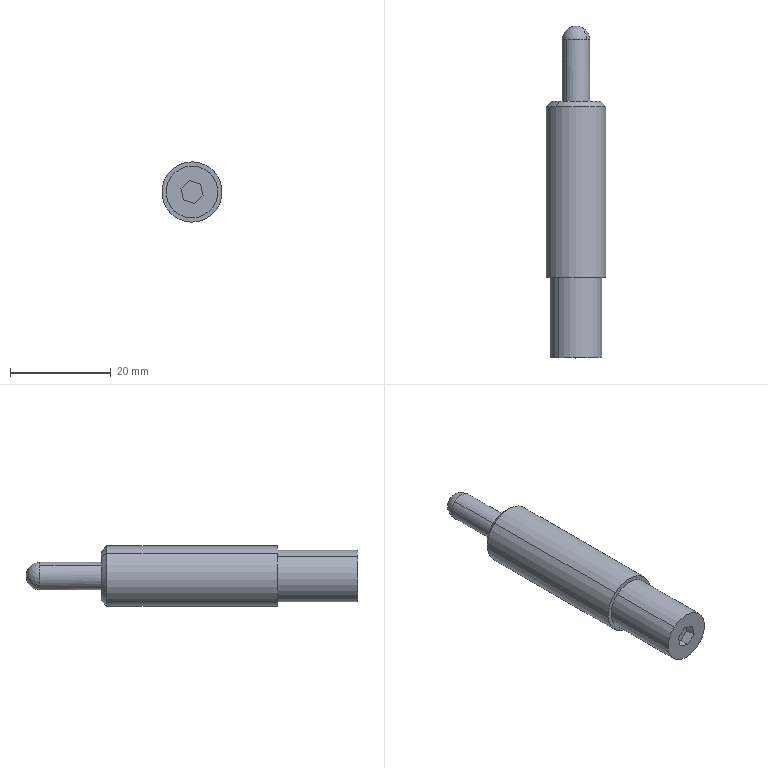Component | SolidWorks | ZAP07-M12-H15-1 | 1 solid | 20 faces | box 12 x 66 x 12 mm | volume 5565 mm3 | plane 10 | cylinder 6 | cone 2 | sphere 2 | commonest cylinder face diameters 10.25 x2 5.5 x2 12 x2
STEP:
#1=COLOUR_RGB('',0.7922,0.8196,0.9333);
#2=FILL_AREA_STYLE_COLOUR('',#1);
#3=FILL_AREA_STYLE('',(#2));
#4=SURFACE_STYLE_FILL_AREA(#3);
#5=SURFACE_SIDE_STYLE('',(#4));
#6=SURFACE_STYLE_USAGE(.BOTH.,#5);
#7=PRESENTATION_STYLE_ASSIGNMENT((#6));
#8=CARTESIAN_POINT('',(-1.631,1.033,9.185));
#9=VERTEX_POINT('',#8);
#10=CARTESIAN_POINT('',(-1.364,1.033,8.882));
#11=VERTEX_POINT('',#10);
#12=CARTESIAN_POINT('',(-1.497,1.033,9.033));
#13=DIRECTION('',(0.,1.,-0.));
#14=DIRECTION('',(-0.6601,0.,0.7512));
#15=AXIS2_PLACEMENT_3D('',#12,#13,#14);
#16=CIRCLE('',#15,0.2018);
#17=EDGE_CURVE('',#9,#11,#16,.T.);
#18=ORIENTED_EDGE('',*,*,#17,.T.);
#19=CARTESIAN_POINT('',(-1.364,1.663,8.882));
#20=VERTEX_POINT('',#19);
#21=CARTESIAN_POINT('',(-1.364,-0.9744,8.882));
#22=DIRECTION('',(0.,1.,-0.));
#23=VECTOR('',#22,39.37);
#24=LINE('',#21,#23);
#25=EDGE_CURVE('',#11,#20,#24,.T.);
#26=ORIENTED_EDGE('',*,*,#25,.T.);
#27=CARTESIAN_POINT('',(-1.631,1.663,9.185));
#28=VERTEX_POINT('',#27);
#29=CARTESIAN_POINT('',(-1.497,1.663,9.033));
#30=DIRECTION('',(0.,1.,-0.));
#31=DIRECTION('',(-0.6601,0.,0.7512));
#32=AXIS2_PLACEMENT_3D('',#29,#30,#31);
#33=CIRCLE('',#32,0.2018);
#34=EDGE_CURVE('',#28,#20,#33,.T.);
#35=ORIENTED_EDGE('',*,*,#34,.F.);
#36=CARTESIAN_POINT('',(-1.631,-0.9744,9.185));
#37=DIRECTION('',(0.,1.,-0.));
#38=VECTOR('',#37,39.37);
#39=LINE('',#36,#38);
#40=EDGE_CURVE('',#9,#28,#39,.T.);
#41=ORIENTED_EDGE('',*,*,#40,.F.);
#42=EDGE_LOOP('',(#18,#26,#35,#41));
#43=FACE_OUTER_BOUND('',#42,.T.);
#44=CARTESIAN_POINT('',(-1.497,-0.9744,9.033));
#45=DIRECTION('',(0.,1.,-0.));
#46=DIRECTION('',(-0.6601,0.,0.7512));
#47=AXIS2_PLACEMENT_3D('',#44,#45,#46);
#48=CYLINDRICAL_SURFACE('',#47,0.2018);
#49=ADVANCED_FACE('',(#43),#48,.T.);
#50=CARTESIAN_POINT('',(-1.626,3.041,9.179));
#51=VERTEX_POINT('',#50);
#52=CARTESIAN_POINT('',(-1.369,3.041,8.887));
#53=VERTEX_POINT('',#52);
#54=CARTESIAN_POINT('',(-1.497,3.041,9.033));
#55=DIRECTION('',(0.,1.,-0.));
#56=DIRECTION('',(-0.6601,0.,0.7512));
#57=AXIS2_PLACEMENT_3D('',#54,#55,#56);
#58=CIRCLE('',#57,0.194);
#59=EDGE_CURVE('',#51,#53,#58,.T.);
#60=ORIENTED_EDGE('',*,*,#59,.F.);
#61=CARTESIAN_POINT('',(-1.653,2.999,9.211));
#62=VERTEX_POINT('',#61);
#63=CARTESIAN_POINT('',(-1.653,2.999,9.211));
#64=DIRECTION('',(-0.4668,-0.7071,0.5311));
#65=VECTOR('',#64,39.37);
#66=LINE('',#63,#65);
#67=EDGE_CURVE('',#51,#62,#66,.T.);
#68=ORIENTED_EDGE('',*,*,#67,.T.);
#69=CARTESIAN_POINT('',(-1.342,2.999,8.856));
#70=VERTEX_POINT('',#69);
#71=CARTESIAN_POINT('',(-1.497,2.999,9.033));
#72=DIRECTION('',(0.,1.,-0.));
#73=DIRECTION('',(-0.6601,0.,0.7512));
#74=AXIS2_PLACEMENT_3D('',#71,#72,#73);
#75=CIRCLE('',#74,0.2362);
#76=EDGE_CURVE('',#62,#70,#75,.T.);
#77=ORIENTED_EDGE('',*,*,#76,.T.);
#78=CARTESIAN_POINT('',(-1.342,2.999,8.856));
#79=DIRECTION('',(0.4668,-0.7071,-0.5311));
#80=VECTOR('',#79,39.37);
#81=LINE('',#78,#80);
#82=EDGE_CURVE('',#53,#70,#81,.T.);
#83=ORIENTED_EDGE('',*,*,#82,.F.);
#84=EDGE_LOOP('',(#60,#68,#77,#83));
#85=FACE_OUTER_BOUND('',#84,.T.);
#86=CARTESIAN_POINT('',(-1.497,2.999,9.033));
#87=DIRECTION('',(-0.,-1.,0.));
#88=DIRECTION('',(0.6601,-0.,-0.7512));
#89=AXIS2_PLACEMENT_3D('',#86,#87,#88);
#90=CONICAL_SURFACE('',#89,0.2362,0.7854);
#91=ADVANCED_FACE('',(#85),#90,.T.);
#92=CARTESIAN_POINT('',(-1.569,3.041,9.114));
#93=VERTEX_POINT('',#92);
#94=CARTESIAN_POINT('',(-1.426,3.041,8.952));
#95=VERTEX_POINT('',#94);
#96=CARTESIAN_POINT('',(-1.497,3.041,9.033));
#97=DIRECTION('',(0.,1.,-0.));
#98=DIRECTION('',(-0.6601,0.,0.7512));
#99=AXIS2_PLACEMENT_3D('',#96,#97,#98);
#100=CIRCLE('',#99,0.1083);
#101=EDGE_CURVE('',#93,#95,#100,.T.);
#102=ORIENTED_EDGE('',*,*,#101,.T.);
#103=CARTESIAN_POINT('',(-1.426,3.524,8.952));
#104=VERTEX_POINT('',#103);
#105=CARTESIAN_POINT('',(-1.426,-0.9744,8.952));
#106=DIRECTION('',(0.,1.,-0.));
#107=VECTOR('',#106,39.37);
#108=LINE('',#105,#107);
#109=EDGE_CURVE('',#95,#104,#108,.T.);
#110=ORIENTED_EDGE('',*,*,#109,.T.);
#111=CARTESIAN_POINT('',(-1.416,3.524,9.105));
#112=VERTEX_POINT('',#111);
#113=CARTESIAN_POINT('',(-1.497,3.524,9.033));
#114=DIRECTION('',(0.,1.,-0.));
#115=DIRECTION('',(-0.6601,0.,0.7512));
#116=AXIS2_PLACEMENT_3D('',#113,#114,#115);
#117=CIRCLE('',#116,0.1083);
#118=EDGE_CURVE('',#112,#104,#117,.T.);
#119=ORIENTED_EDGE('',*,*,#118,.F.);
#120=CARTESIAN_POINT('',(-1.569,3.524,9.114));
#121=VERTEX_POINT('',#120);
#122=CARTESIAN_POINT('',(-1.497,3.524,9.033));
#123=DIRECTION('',(0.,1.,-0.));
#124=DIRECTION('',(-0.6601,0.,0.7512));
#125=AXIS2_PLACEMENT_3D('',#122,#123,#124);
#126=CIRCLE('',#125,0.1083);
#127=EDGE_CURVE('',#121,#112,#126,.T.);
#128=ORIENTED_EDGE('',*,*,#127,.F.);
#129=CARTESIAN_POINT('',(-1.569,-0.9744,9.114));
#130=DIRECTION('',(0.,1.,-0.));
#131=VECTOR('',#130,39.37);
#132=LINE('',#129,#131);
#133=EDGE_CURVE('',#93,#121,#132,.T.);
#134=ORIENTED_EDGE('',*,*,#133,.F.);
#135=EDGE_LOOP('',(#102,#110,#119,#128,#134));
#136=FACE_OUTER_BOUND('',#135,.T.);
#137=CARTESIAN_POINT('',(-1.497,-0.9744,9.033));
#138=DIRECTION('',(0.,1.,-0.));
#139=DIRECTION('',(-0.6601,0.,0.7512));
#140=AXIS2_PLACEMENT_3D('',#137,#138,#139);
#141=CYLINDRICAL_SURFACE('',#140,0.1083);
#142=ADVANCED_FACE('',(#136),#141,.T.);
#143=ORIENTED_EDGE('',*,*,#118,.T.);
#144=CARTESIAN_POINT('',(-1.579,3.524,8.962));
#145=VERTEX_POINT('',#144);
#146=CARTESIAN_POINT('',(-1.497,3.524,9.033));
#147=DIRECTION('',(0.,1.,-0.));
#148=DIRECTION('',(-0.6601,0.,0.7512));
#149=AXIS2_PLACEMENT_3D('',#146,#147,#148);
#150=CIRCLE('',#149,0.1083);
#151=EDGE_CURVE('',#104,#145,#150,.T.);
#152=ORIENTED_EDGE('',*,*,#151,.T.);
#153=CARTESIAN_POINT('',(-1.497,3.632,9.033));
#154=VERTEX_POINT('',#153);
#155=CARTESIAN_POINT('',(-1.497,3.524,9.033));
#156=DIRECTION('',(0.6601,-0.,-0.7512));
#157=DIRECTION('',(-0.7512,0.,-0.6601));
#158=AXIS2_PLACEMENT_3D('',#155,#156,#157);
#159=CIRCLE('',#158,0.1083);
#160=EDGE_CURVE('',#145,#154,#159,.T.);
#161=ORIENTED_EDGE('',*,*,#160,.T.);
#162=CARTESIAN_POINT('',(-1.497,3.524,9.033));
#163=DIRECTION('',(-0.6601,0.,0.7512));
#164=DIRECTION('',(0.7512,0.,0.6601));
#165=AXIS2_PLACEMENT_3D('',#162,#163,#164);
#166=CIRCLE('',#165,0.1083);
#167=EDGE_CURVE('',#112,#154,#166,.T.);
#168=ORIENTED_EDGE('',*,*,#167,.F.);
#169=EDGE_LOOP('',(#143,#152,#161,#168));
#170=FACE_OUTER_BOUND('',#169,.T.);
#171=CARTESIAN_POINT('',(-1.497,3.524,9.033));
#172=DIRECTION('',(0.6601,-0.,-0.7512));
#173=DIRECTION('',(0.7512,-0.,0.6601));
#174=AXIS2_PLACEMENT_3D('',#171,#172,#173);
#175=SPHERICAL_SURFACE('',#174,0.1083);
#176=ADVANCED_FACE('',(#170),#175,.T.);
#177=CARTESIAN_POINT('',(-1.653,1.663,9.211));
#178=VERTEX_POINT('',#177);
#179=CARTESIAN_POINT('',(-1.342,1.663,8.856));
#180=VERTEX_POINT('',#179);
#181=CARTESIAN_POINT('',(-1.497,1.663,9.033));
#182=DIRECTION('',(0.,1.,-0.));
#183=DIRECTION('',(-0.6601,0.,0.7512));
#184=AXIS2_PLACEMENT_3D('',#181,#182,#183);
#185=CIRCLE('',#184,0.2362);
#186=EDGE_CURVE('',#178,#180,#185,.T.);
#187=ORIENTED_EDGE('',*,*,#186,.T.);
#188=CARTESIAN_POINT('',(-1.342,-0.9744,8.856));
#189=DIRECTION('',(0.,1.,-0.));
#190=VECTOR('',#189,39.37);
#191=LINE('',#188,#190);
#192=EDGE_CURVE('',#180,#70,#191,.T.);
#193=ORIENTED_EDGE('',*,*,#192,.T.);
#194=ORIENTED_EDGE('',*,*,#76,.F.);
#195=CARTESIAN_POINT('',(-1.653,-0.9744,9.211));
#196=DIRECTION('',(0.,1.,-0.));
#197=VECTOR('',#196,39.37);
#198=LINE('',#195,#197);
#199=EDGE_CURVE('',#178,#62,#198,.T.);
#200=ORIENTED_EDGE('',*,*,#199,.F.);
#201=EDGE_LOOP('',(#187,#193,#194,#200));
#202=FACE_OUTER_BOUND('',#201,.T.);
#203=CARTESIAN_POINT('',(-1.497,-0.9744,9.033));
#204=DIRECTION('',(0.,1.,-0.));
#205=DIRECTION('',(-0.6601,0.,0.7512));
#206=AXIS2_PLACEMENT_3D('',#203,#204,#205);
#207=CYLINDRICAL_SURFACE('',#206,0.2362);
#208=ADVANCED_FACE('',(#202),#207,.T.);
#209=ORIENTED_EDGE('',*,*,#192,.F.);
#210=CARTESIAN_POINT('',(-1.497,1.663,9.033));
#211=DIRECTION('',(0.,1.,-0.));
#212=DIRECTION('',(-0.6601,0.,0.7512));
#213=AXIS2_PLACEMENT_3D('',#210,#211,#212);
#214=CIRCLE('',#213,0.2362);
#215=EDGE_CURVE('',#180,#178,#214,.T.);
#216=ORIENTED_EDGE('',*,*,#215,.T.);
#217=ORIENTED_EDGE('',*,*,#199,.T.);
#218=CARTESIAN_POINT('',(-1.497,2.999,9.033));
#219=DIRECTION('',(0.,1.,-0.));
#220=DIRECTION('',(-0.6601,0.,0.7512));
#221=AXIS2_PLACEMENT_3D('',#218,#219,#220);
#222=CIRCLE('',#221,0.2362);
#223=EDGE_CURVE('',#70,#62,#222,.T.);
#224=ORIENTED_EDGE('',*,*,#223,.F.);
#225=EDGE_LOOP('',(#209,#216,#217,#224));
#226=FACE_OUTER_BOUND('',#225,.T.);
#227=CARTESIAN_POINT('',(-1.497,-0.9744,9.033));
#228=DIRECTION('',(0.,1.,-0.));
#229=DIRECTION('',(-0.6601,0.,0.7512));
#230=AXIS2_PLACEMENT_3D('',#227,#228,#229);
#231=CYLINDRICAL_SURFACE('',#230,0.2362);
#232=ADVANCED_FACE('',(#226),#231,.T.);
#233=ORIENTED_EDGE('',*,*,#160,.F.);
#234=CARTESIAN_POINT('',(-1.497,3.524,9.033));
#235=DIRECTION('',(0.,1.,-0.));
#236=DIRECTION('',(-0.6601,0.,0.7512));
#237=AXIS2_PLACEMENT_3D('',#234,#235,#236);
#238=CIRCLE('',#237,0.1083);
#239=EDGE_CURVE('',#145,#121,#238,.T.);
#240=ORIENTED_EDGE('',*,*,#239,.T.);
#241=ORIENTED_EDGE('',*,*,#127,.T.);
#242=ORIENTED_EDGE('',*,*,#167,.T.);
#243=EDGE_LOOP('',(#233,#240,#241,#242));
#244=FACE_OUTER_BOUND('',#243,.T.);
#245=CARTESIAN_POINT('',(-1.497,3.524,9.033));
#246=DIRECTION('',(0.6601,-0.,-0.7512));
#247=DIRECTION('',(0.7512,-0.,0.6601));
#248=AXIS2_PLACEMENT_3D('',#245,#246,#247);
#249=SPHERICAL_SURFACE('',#248,0.1083);
#250=ADVANCED_FACE('',(#244),#249,.T.);
#251=ORIENTED_EDGE('',*,*,#109,.F.);
#252=CARTESIAN_POINT('',(-1.497,3.041,9.033));
#253=DIRECTION('',(0.,1.,-0.));
#254=DIRECTION('',(-0.6601,0.,0.7512));
#255=AXIS2_PLACEMENT_3D('',#252,#253,#254);
#256=CIRCLE('',#255,0.1083);
#257=EDGE_CURVE('',#95,#93,#256,.T.);
#258=ORIENTED_EDGE('',*,*,#257,.T.);
#259=ORIENTED_EDGE('',*,*,#133,.T.);
#260=ORIENTED_EDGE('',*,*,#239,.F.);
#261=ORIENTED_EDGE('',*,*,#151,.F.);
#262=EDGE_LOOP('',(#251,#258,#259,#260,#261));
#263=FACE_OUTER_BOUND('',#262,.T.);
#264=CARTESIAN_POINT('',(-1.497,-0.9744,9.033));
#265=DIRECTION('',(0.,1.,-0.));
#266=DIRECTION('',(-0.6601,0.,0.7512));
#267=AXIS2_PLACEMENT_3D('',#264,#265,#266);
#268=CYLINDRICAL_SURFACE('',#267,0.1083);
#269=ADVANCED_FACE('',(#263),#268,.T.);
#270=ORIENTED_EDGE('',*,*,#101,.F.);
#271=ORIENTED_EDGE('',*,*,#257,.F.);
#272=EDGE_LOOP('',(#270,#271));
#273=FACE_BOUND('',#272,.T.);
#274=CARTESIAN_POINT('',(-1.497,3.041,9.033));
#275=DIRECTION('',(0.,1.,-0.));
#276=DIRECTION('',(-0.6601,0.,0.7512));
#277=AXIS2_PLACEMENT_3D('',#274,#275,#276);
#278=CIRCLE('',#277,0.194);
#279=EDGE_CURVE('',#53,#51,#278,.T.);
#280=ORIENTED_EDGE('',*,*,#279,.T.);
#281=ORIENTED_EDGE('',*,*,#59,.T.);
#282=EDGE_LOOP('',(#280,#281));
#283=FACE_OUTER_BOUND('',#282,.T.);
#284=CARTESIAN_POINT('',(-1.416,3.041,9.105));
#285=DIRECTION('',(-0.,-1.,0.));
#286=DIRECTION('',(0.6601,-0.,-0.7512));
#287=AXIS2_PLACEMENT_3D('',#284,#285,#286);
#288=PLANE('',#287);
#289=ADVANCED_FACE('',(#273,#283),#288,.F.);
#290=ORIENTED_EDGE('',*,*,#67,.F.);
#291=ORIENTED_EDGE('',*,*,#279,.F.);
#292=ORIENTED_EDGE('',*,*,#82,.T.);
#293=ORIENTED_EDGE('',*,*,#223,.T.);
#294=EDGE_LOOP('',(#290,#291,#292,#293));
#295=FACE_OUTER_BOUND('',#294,.T.);
#296=CARTESIAN_POINT('',(-1.497,2.999,9.033));
#297=DIRECTION('',(-0.,-1.,0.));
#298=DIRECTION('',(0.6601,-0.,-0.7512));
#299=AXIS2_PLACEMENT_3D('',#296,#297,#298);
#300=CONICAL_SURFACE('',#299,0.2362,0.7854);
#301=ADVANCED_FACE('',(#295),#300,.T.);
#302=ORIENTED_EDGE('',*,*,#34,.T.);
#303=CARTESIAN_POINT('',(-1.497,1.663,9.033));
#304=DIRECTION('',(0.,1.,-0.));
#305=DIRECTION('',(-0.6601,0.,0.7512));
#306=AXIS2_PLACEMENT_3D('',#303,#304,#305);
#307=CIRCLE('',#306,0.2018);
#308=EDGE_CURVE('',#20,#28,#307,.T.);
#309=ORIENTED_EDGE('',*,*,#308,.T.);
#310=EDGE_LOOP('',(#302,#309));
#311=FACE_BOUND('',#310,.T.);
#312=ORIENTED_EDGE('',*,*,#186,.F.);
#313=ORIENTED_EDGE('',*,*,#215,.F.);
#314=EDGE_LOOP('',(#312,#313));
#315=FACE_OUTER_BOUND('',#314,.T.);
#316=CARTESIAN_POINT('',(-1.32,1.663,9.189));
#317=DIRECTION('',(-0.,-1.,0.));
#318=DIRECTION('',(0.6601,-0.,-0.7512));
#319=AXIS2_PLACEMENT_3D('',#316,#317,#318);
#320=PLANE('',#319);
#321=ADVANCED_FACE('',(#311,#315),#320,.T.);
#322=ORIENTED_EDGE('',*,*,#25,.F.);
#323=CARTESIAN_POINT('',(-1.497,1.033,9.033));
#324=DIRECTION('',(0.,1.,-0.));
#325=DIRECTION('',(-0.6601,0.,0.7512));
#326=AXIS2_PLACEMENT_3D('',#323,#324,#325);
#327=CIRCLE('',#326,0.2018);
#328=EDGE_CURVE('',#11,#9,#327,.T.);
#329=ORIENTED_EDGE('',*,*,#328,.T.);
#330=ORIENTED_EDGE('',*,*,#40,.T.);
#331=ORIENTED_EDGE('',*,*,#308,.F.);
#332=EDGE_LOOP('',(#322,#329,#330,#331));
#333=FACE_OUTER_BOUND('',#332,.T.);
#334=CARTESIAN_POINT('',(-1.497,-0.9744,9.033));
#335=DIRECTION('',(0.,1.,-0.));
#336=DIRECTION('',(-0.6601,0.,0.7512));
#337=AXIS2_PLACEMENT_3D('',#334,#335,#336);
#338=CYLINDRICAL_SURFACE('',#337,0.2018);
#339=ADVANCED_FACE('',(#333),#338,.T.);
#340=CARTESIAN_POINT('',(-1.584,1.033,9.062));
#341=VERTEX_POINT('',#340);
#342=CARTESIAN_POINT('',(-1.566,1.033,8.973));
#343=VERTEX_POINT('',#342);
#344=CARTESIAN_POINT('',(-1.584,1.033,9.062));
#345=DIRECTION('',(0.1961,-0.,-0.9806));
#346=VECTOR('',#345,39.37);
#347=LINE('',#344,#346);
#348=EDGE_CURVE('',#341,#343,#347,.T.);
#349=ORIENTED_EDGE('',*,*,#348,.F.);
#350=CARTESIAN_POINT('',(-1.515,1.033,9.122));
#351=VERTEX_POINT('',#350);
#352=CARTESIAN_POINT('',(-1.515,1.033,9.122));
#353=DIRECTION('',(-0.7512,0.,-0.6601));
#354=VECTOR('',#353,39.37);
#355=LINE('',#352,#354);
#356=EDGE_CURVE('',#351,#341,#355,.T.);
#357=ORIENTED_EDGE('',*,*,#356,.F.);
#358=CARTESIAN_POINT('',(-1.429,1.033,9.093));
#359=VERTEX_POINT('',#358);
#360=CARTESIAN_POINT('',(-1.429,1.033,9.093));
#361=DIRECTION('',(-0.9473,0.,0.3205));
#362=VECTOR('',#361,39.37);
#363=LINE('',#360,#362);
#364=EDGE_CURVE('',#359,#351,#363,.T.);
#365=ORIENTED_EDGE('',*,*,#364,.F.);
#366=CARTESIAN_POINT('',(-1.411,1.033,9.004));
#367=VERTEX_POINT('',#366);
#368=CARTESIAN_POINT('',(-1.411,1.033,9.004));
#369=DIRECTION('',(-0.1961,0.,0.9806));
#370=VECTOR('',#369,39.37);
#371=LINE('',#368,#370);
#372=EDGE_CURVE('',#367,#359,#371,.T.);
#373=ORIENTED_EDGE('',*,*,#372,.F.);
#374=CARTESIAN_POINT('',(-1.48,1.033,8.944));
#375=VERTEX_POINT('',#374);
#376=CARTESIAN_POINT('',(-1.48,1.033,8.944));
#377=DIRECTION('',(0.7512,-0.,0.6601));
#378=VECTOR('',#377,39.37);
#379=LINE('',#376,#378);
#380=EDGE_CURVE('',#375,#367,#379,.T.);
#381=ORIENTED_EDGE('',*,*,#380,.F.);
#382=CARTESIAN_POINT('',(-1.566,1.033,8.973));
#383=DIRECTION('',(0.9473,-0.,-0.3205));
#384=VECTOR('',#383,39.37);
#385=LINE('',#382,#384);
#386=EDGE_CURVE('',#343,#375,#385,.T.);
#387=ORIENTED_EDGE('',*,*,#386,.F.);
#388=EDGE_LOOP('',(#349,#357,#365,#373,#381,#387));
#389=FACE_BOUND('',#388,.T.);
#390=ORIENTED_EDGE('',*,*,#17,.F.);
#391=ORIENTED_EDGE('',*,*,#328,.F.);
#392=EDGE_LOOP('',(#390,#391));
#393=FACE_OUTER_BOUND('',#392,.T.);
#394=CARTESIAN_POINT('',(-1.333,1.033,9.178));
#395=DIRECTION('',(0.,1.,-0.));
#396=DIRECTION('',(-0.6601,0.,0.7512));
#397=AXIS2_PLACEMENT_3D('',#394,#395,#396);
#398=PLANE('',#397);
#399=ADVANCED_FACE('',(#389,#393),#398,.F.);
#400=ORIENTED_EDGE('',*,*,#356,.T.);
#401=CARTESIAN_POINT('',(-1.584,1.112,9.062));
#402=VERTEX_POINT('',#401);
#403=CARTESIAN_POINT('',(-1.584,1.112,9.062));
#404=DIRECTION('',(-0.,-1.,0.));
#405=VECTOR('',#404,39.37);
#406=LINE('',#403,#405);
#407=EDGE_CURVE('',#402,#341,#406,.T.);
#408=ORIENTED_EDGE('',*,*,#407,.F.);
#409=CARTESIAN_POINT('',(-1.515,1.112,9.122));
#410=VERTEX_POINT('',#409);
#411=CARTESIAN_POINT('',(-1.515,1.112,9.122));
#412=DIRECTION('',(-0.7512,0.,-0.6601));
#413=VECTOR('',#412,39.37);
#414=LINE('',#411,#413);
#415=EDGE_CURVE('',#410,#402,#414,.T.);
#416=ORIENTED_EDGE('',*,*,#415,.F.);
#417=CARTESIAN_POINT('',(-1.515,1.112,9.122));
#418=DIRECTION('',(-0.,-1.,0.));
#419=VECTOR('',#418,39.37);
#420=LINE('',#417,#419);
#421=EDGE_CURVE('',#410,#351,#420,.T.);
#422=ORIENTED_EDGE('',*,*,#421,.T.);
#423=EDGE_LOOP('',(#400,#408,#416,#422));
#424=FACE_OUTER_BOUND('',#423,.T.);
#425=CARTESIAN_POINT('',(-1.515,1.112,9.122));
#426=DIRECTION('',(-0.6601,0.,0.7512));
#427=DIRECTION('',(-0.,-1.,0.));
#428=AXIS2_PLACEMENT_3D('',#425,#426,#427);
#429=PLANE('',#428);
#430=ADVANCED_FACE('',(#424),#429,.F.);
#431=ORIENTED_EDGE('',*,*,#364,.T.);
#432=ORIENTED_EDGE('',*,*,#421,.F.);
#433=CARTESIAN_POINT('',(-1.429,1.112,9.093));
#434=VERTEX_POINT('',#433);
#435=CARTESIAN_POINT('',(-1.429,1.112,9.093));
#436=DIRECTION('',(-0.9473,0.,0.3205));
#437=VECTOR('',#436,39.37);
#438=LINE('',#435,#437);
#439=EDGE_CURVE('',#434,#410,#438,.T.);
#440=ORIENTED_EDGE('',*,*,#439,.F.);
#441=CARTESIAN_POINT('',(-1.429,1.112,9.093));
#442=DIRECTION('',(-0.,-1.,0.));
#443=VECTOR('',#442,39.37);
#444=LINE('',#441,#443);
#445=EDGE_CURVE('',#434,#359,#444,.T.);
#446=ORIENTED_EDGE('',*,*,#445,.T.);
#447=EDGE_LOOP('',(#431,#432,#440,#446));
#448=FACE_OUTER_BOUND('',#447,.T.);
#449=CARTESIAN_POINT('',(-1.429,1.112,9.093));
#450=DIRECTION('',(0.3205,-0.,0.9473));
#451=DIRECTION('',(-0.9473,0.,0.3205));
#452=AXIS2_PLACEMENT_3D('',#449,#450,#451);
#453=PLANE('',#452);
#454=ADVANCED_FACE('',(#448),#453,.F.);
#455=ORIENTED_EDGE('',*,*,#372,.T.);
#456=ORIENTED_EDGE('',*,*,#445,.F.);
#457=CARTESIAN_POINT('',(-1.411,1.112,9.004));
#458=VERTEX_POINT('',#457);
#459=CARTESIAN_POINT('',(-1.411,1.112,9.004));
#460=DIRECTION('',(-0.1961,0.,0.9806));
#461=VECTOR('',#460,39.37);
#462=LINE('',#459,#461);
#463=EDGE_CURVE('',#458,#434,#462,.T.);
#464=ORIENTED_EDGE('',*,*,#463,.F.);
#465=CARTESIAN_POINT('',(-1.411,1.112,9.004));
#466=DIRECTION('',(-0.,-1.,0.));
#467=VECTOR('',#466,39.37);
#468=LINE('',#465,#467);
#469=EDGE_CURVE('',#458,#367,#468,.T.);
#470=ORIENTED_EDGE('',*,*,#469,.T.);
#471=EDGE_LOOP('',(#455,#456,#464,#470));
#472=FACE_OUTER_BOUND('',#471,.T.);
#473=CARTESIAN_POINT('',(-1.411,1.112,9.004));
#474=DIRECTION('',(0.9806,-0.,0.1961));
#475=DIRECTION('',(-0.1961,0.,0.9806));
#476=AXIS2_PLACEMENT_3D('',#473,#474,#475);
#477=PLANE('',#476);
#478=ADVANCED_FACE('',(#472),#477,.F.);
#479=ORIENTED_EDGE('',*,*,#380,.T.);
#480=ORIENTED_EDGE('',*,*,#469,.F.);
#481=CARTESIAN_POINT('',(-1.48,1.112,8.944));
#482=VERTEX_POINT('',#481);
#483=CARTESIAN_POINT('',(-1.48,1.112,8.944));
#484=DIRECTION('',(0.7512,-0.,0.6601));
#485=VECTOR('',#484,39.37);
#486=LINE('',#483,#485);
#487=EDGE_CURVE('',#482,#458,#486,.T.);
#488=ORIENTED_EDGE('',*,*,#487,.F.);
#489=CARTESIAN_POINT('',(-1.48,1.112,8.944));
#490=DIRECTION('',(-0.,-1.,0.));
#491=VECTOR('',#490,39.37);
#492=LINE('',#489,#491);
#493=EDGE_CURVE('',#482,#375,#492,.T.);
#494=ORIENTED_EDGE('',*,*,#493,.T.);
#495=EDGE_LOOP('',(#479,#480,#488,#494));
#496=FACE_OUTER_BOUND('',#495,.T.);
#497=CARTESIAN_POINT('',(-1.48,1.112,8.944));
#498=DIRECTION('',(0.6601,-0.,-0.7512));
#499=DIRECTION('',(0.,1.,-0.));
#500=AXIS2_PLACEMENT_3D('',#497,#498,#499);
#501=PLANE('',#500);
#502=ADVANCED_FACE('',(#496),#501,.F.);
#503=ORIENTED_EDGE('',*,*,#386,.T.);
#504=ORIENTED_EDGE('',*,*,#493,.F.);
#505=CARTESIAN_POINT('',(-1.566,1.112,8.973));
#506=VERTEX_POINT('',#505);
#507=CARTESIAN_POINT('',(-1.566,1.112,8.973));
#508=DIRECTION('',(0.9473,-0.,-0.3205));
#509=VECTOR('',#508,39.37);
#510=LINE('',#507,#509);
#511=EDGE_CURVE('',#506,#482,#510,.T.);
#512=ORIENTED_EDGE('',*,*,#511,.F.);
#513=CARTESIAN_POINT('',(-1.566,1.112,8.973));
#514=DIRECTION('',(-0.,-1.,0.));
#515=VECTOR('',#514,39.37);
#516=LINE('',#513,#515);
#517=EDGE_CURVE('',#506,#343,#516,.T.);
#518=ORIENTED_EDGE('',*,*,#517,.T.);
#519=EDGE_LOOP('',(#503,#504,#512,#518));
#520=FACE_OUTER_BOUND('',#519,.T.);
#521=CARTESIAN_POINT('',(-1.566,1.112,8.973));
#522=DIRECTION('',(-0.3205,0.,-0.9473));
#523=DIRECTION('',(0.9473,-0.,-0.3205));
#524=AXIS2_PLACEMENT_3D('',#521,#522,#523);
#525=PLANE('',#524);
#526=ADVANCED_FACE('',(#520),#525,.F.);
#527=ORIENTED_EDGE('',*,*,#348,.T.);
#528=ORIENTED_EDGE('',*,*,#517,.F.);
#529=CARTESIAN_POINT('',(-1.584,1.112,9.062));
#530=DIRECTION('',(0.1961,-0.,-0.9806));
#531=VECTOR('',#530,39.37);
#532=LINE('',#529,#531);
#533=EDGE_CURVE('',#402,#506,#532,.T.);
#534=ORIENTED_EDGE('',*,*,#533,.F.);
#535=ORIENTED_EDGE('',*,*,#407,.T.);
#536=EDGE_LOOP('',(#527,#528,#534,#535));
#537=FACE_OUTER_BOUND('',#536,.T.);
#538=CARTESIAN_POINT('',(-1.584,1.112,9.062));
#539=DIRECTION('',(-0.9806,0.,-0.1961));
#540=DIRECTION('',(0.1961,-0.,-0.9806));
#541=AXIS2_PLACEMENT_3D('',#538,#539,#540);
#542=PLANE('',#541);
#543=ADVANCED_FACE('',(#537),#542,.F.);
#544=ORIENTED_EDGE('',*,*,#415,.T.);
#545=ORIENTED_EDGE('',*,*,#533,.T.);
#546=ORIENTED_EDGE('',*,*,#511,.T.);
#547=ORIENTED_EDGE('',*,*,#487,.T.);
#548=ORIENTED_EDGE('',*,*,#463,.T.);
#549=ORIENTED_EDGE('',*,*,#439,.T.);
#550=EDGE_LOOP('',(#544,#545,#546,#547,#548,#549));
#551=FACE_OUTER_BOUND('',#550,.T.);
#552=CARTESIAN_POINT('',(-1.497,1.112,9.033));
#553=DIRECTION('',(-0.,-1.,0.));
#554=DIRECTION('',(0.6601,-0.,-0.7512));
#555=AXIS2_PLACEMENT_3D('',#552,#553,#554);
#556=PLANE('',#555);
#557=ADVANCED_FACE('',(#551),#556,.T.);
#558=CLOSED_SHELL('',(#49,#91,#142,#176,#208,#232,#250,#269,#289,#301,#321,#339,#399,#430,#454,#478,#502,#526,#543,#557));
#559=MANIFOLD_SOLID_BREP('',#558);
#560=STYLED_ITEM('',(#7),#559);
#561=PRESENTATION_LAYER_ASSIGNMENT('','',(#560));
#562=CARTESIAN_POINT('',(0.,0.,0.));
#563=DIRECTION('',(0.,0.,1.));
#564=DIRECTION('',(1.,0.,0.));
#565=AXIS2_PLACEMENT_3D('',#562,#563,#564);
#566=(LENGTH_UNIT()NAMED_UNIT(*)SI_UNIT($,.METRE.));
#567=LENGTH_MEASURE_WITH_UNIT(LENGTH_MEASURE(0.0254),#566);
#568=DIMENSIONAL_EXPONENTS(1.,0.,0.,0.,0.,0.,0.);
#569=(CONVERSION_BASED_UNIT('',#567)LENGTH_UNIT()NAMED_UNIT(#568));
#570=UNCERTAINTY_MEASURE_WITH_UNIT(LENGTH_MEASURE(0.00001),#569,'','');
#571=(NAMED_UNIT(*)PLANE_ANGLE_UNIT()SI_UNIT($,.RADIAN.));
#572=(NAMED_UNIT(*)SI_UNIT($,.STERADIAN.)SOLID_ANGLE_UNIT());
#573=(GEOMETRIC_REPRESENTATION_CONTEXT(3)GLOBAL_UNCERTAINTY_ASSIGNED_CONTEXT((#570))GLOBAL_UNIT_ASSIGNED_CONTEXT((#569,#571,#572))REPRESENTATION_CONTEXT('',''));
#574=ADVANCED_BREP_SHAPE_REPRESENTATION('',(#559,#565),#573);
#575=(LENGTH_UNIT()NAMED_UNIT(*)SI_UNIT($,.METRE.));
#576=LENGTH_MEASURE_WITH_UNIT(LENGTH_MEASURE(0.0254),#575);
#577=DIMENSIONAL_EXPONENTS(1.,0.,0.,0.,0.,0.,0.);
#578=(CONVERSION_BASED_UNIT('',#576)LENGTH_UNIT()NAMED_UNIT(#577));
#579=UNCERTAINTY_MEASURE_WITH_UNIT(LENGTH_MEASURE(0.00001),#578,'','');
#580=(NAMED_UNIT(*)PLANE_ANGLE_UNIT()SI_UNIT($,.RADIAN.));
#581=(NAMED_UNIT(*)SI_UNIT($,.STERADIAN.)SOLID_ANGLE_UNIT());
#582=(GEOMETRIC_REPRESENTATION_CONTEXT(3)GLOBAL_UNCERTAINTY_ASSIGNED_CONTEXT((#579))GLOBAL_UNIT_ASSIGNED_CONTEXT((#578,#580,#581))REPRESENTATION_CONTEXT('',''));
#583=MECHANICAL_DESIGN_GEOMETRIC_PRESENTATION_REPRESENTATION('',(#560),#582);